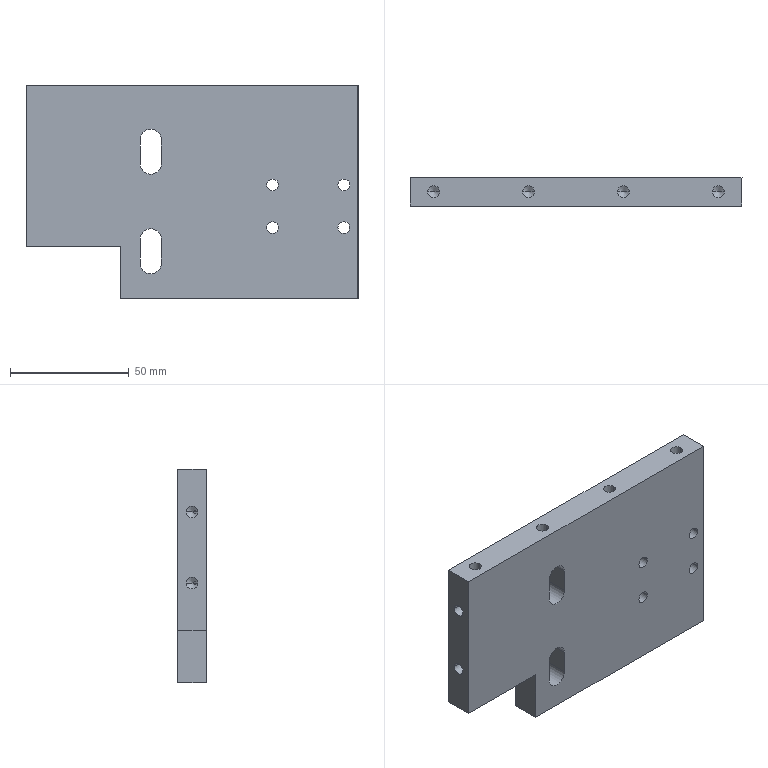Component | SolidWorks | 17081801-804-012A-1 | 1 solid | 72 faces | box 140 x 12 x 90 mm | volume 132790 mm3 | cylinder 36 | cone 24 | plane 12 | commonest cylinder face diameters 5 x32 9 x4 | material Q235
build123d program:
from build123d import *

# Parameters (mm, degrees)
SKETCH1_W                     = 12
SKETCH1_H                     = 90
BOSS_EXTRUDE1_DEPTH           = 40
SKETCH4_W                     = 12
SKETCH4_H                     = 68
BOSS_EXTRUDE2_DEPTH           = 60
M6_TAPPED_HOLE1_D             = 5
M6_TAPPED_HOLE1_DEPTH         = 13
M6_TAPPED_HOLE1_TIP           = 1.502
M6_TAPPED_HOLE2_D             = 5
M6_TAPPED_HOLE2_DEPTH         = 13
M6_TAPPED_HOLE2_TIP           = 1.502
SKETCH10_W                    = 12
SKETCH10_H                    = 22
BOSS_EXTRUDE3_DEPTH           = 20
CUT_EXTRUDE1_DEPTH            = 136.07
M6_TAPPED_HOLE3_D             = 5
M6_TAPPED_HOLE3_DEPTH         = 15
M6_TAPPED_HOLE3_TIP           = 1.502
SIZE_MM_DOWEL_PIN_HOLE1_D     = 5
SIZE_MM_DOWEL_PIN_HOLE1_DEPTH = 10
SIZE_MM_DOWEL_PIN_HOLE1_TIP   = 1.502
M6_TAPPED_HOLE4_D             = 5
M6_TAPPED_HOLE4_DEPTH         = 15
M6_TAPPED_HOLE4_TIP           = 1.502


with BuildPart() as part:
    # Sketch1 → Boss-Extrude1 (new, symmetric)
    with BuildSketch(Plane.XY):
        with Locations((0, 45)):
            Rectangle(SKETCH1_W, SKETCH1_H)
    extrude(amount=BOSS_EXTRUDE1_DEPTH, both=True)

    # Sketch4 → Boss-Extrude2 (add)
    with BuildSketch(Plane(origin=(0, 0, -40), x_dir=(-1, 0, 0), z_dir=(0, 0, -1))):
        with Locations((0, 56)):
            Rectangle(SKETCH4_W, SKETCH4_H)
    extrude(amount=BOSS_EXTRUDE2_DEPTH)

    # M6 Tapped Hole1
    with Locations(Plane(origin=(0, 90, 0), x_dir=(1, 0, 0), z_dir=(0, 1, 0))):
        with Locations((0, -30), (0, 10), (0, 50), (0, 90)):
            Hole(M6_TAPPED_HOLE1_D / 2, depth=M6_TAPPED_HOLE1_DEPTH)
            with Locations((0, 0, -(M6_TAPPED_HOLE1_DEPTH + M6_TAPPED_HOLE1_TIP / 2))):  # 118° drill point
                Cone(0, M6_TAPPED_HOLE1_D / 2, M6_TAPPED_HOLE1_TIP, mode=Mode.SUBTRACT)

    # M6 Tapped Hole2
    with Locations(Plane(origin=(0, 0, -100), x_dir=(-1, 0, 0), z_dir=(0, 0, -1))):
        with Locations((0, 42), (0, 72)):
            Hole(M6_TAPPED_HOLE2_D / 2, depth=M6_TAPPED_HOLE2_DEPTH)
            with Locations((0, 0, -(M6_TAPPED_HOLE2_DEPTH + M6_TAPPED_HOLE2_TIP / 2))):  # 118° drill point
                Cone(0, M6_TAPPED_HOLE2_D / 2, M6_TAPPED_HOLE2_TIP, mode=Mode.SUBTRACT)

    # Sketch10 → Boss-Extrude3 (add)
    with BuildSketch(Plane(origin=(0, 0, -40), x_dir=(-1, 0, 0), z_dir=(0, 0, -1))):
        with Locations((0, 11)):
            Rectangle(SKETCH10_W, SKETCH10_H)
    extrude(amount=BOSS_EXTRUDE3_DEPTH)

    # Sketch11 → Cut-Extrude1 (cut, through all)
    with BuildSketch(Plane(origin=(6, 0, 0), x_dir=(0, 0, -1), z_dir=(1, 0, 0))):
        with BuildLine():
            Line((42.9, 15), (42.9, 25))
            ThreePointArc((42.9, 25), (47.4, 29.5), (51.9, 25))
            Line((51.9, 25), (51.9, 15))
            ThreePointArc((51.9, 15), (47.4, 10.5), (42.9, 15))
        make_face()
        with BuildLine():
            Line((42.9, 57), (42.9, 67))
            ThreePointArc((42.9, 67), (47.4, 71.5), (51.9, 67))
            Line((51.9, 67), (51.9, 57))
            ThreePointArc((51.9, 57), (47.4, 52.5), (42.9, 57))
        make_face()
    extrude(amount=-CUT_EXTRUDE1_DEPTH, mode=Mode.SUBTRACT)

    # M6 Tapped Hole3
    with Locations(Plane(origin=(0, 0, 0), x_dir=(-1, 0, 0), z_dir=(0, -1, 0))):
        with Locations((0, -35), (0, -15), (0, 15), (0, 35)):
            Hole(M6_TAPPED_HOLE3_D / 2, depth=M6_TAPPED_HOLE3_DEPTH)
            with Locations((0, 0, -(M6_TAPPED_HOLE3_DEPTH + M6_TAPPED_HOLE3_TIP / 2))):  # 118° drill point
                Cone(0, M6_TAPPED_HOLE3_D / 2, M6_TAPPED_HOLE3_TIP, mode=Mode.SUBTRACT)

    # Size mm Dowel Pin Hole1
    with Locations(Plane(origin=(0, 0, 0), x_dir=(-1, 0, 0), z_dir=(0, -1, 0))):
        with Locations((0, 25), (0, -25)):
            Hole(SIZE_MM_DOWEL_PIN_HOLE1_D / 2, depth=SIZE_MM_DOWEL_PIN_HOLE1_DEPTH)
            with Locations((0, 0, -(SIZE_MM_DOWEL_PIN_HOLE1_DEPTH + SIZE_MM_DOWEL_PIN_HOLE1_TIP / 2))):  # 118° drill point
                Cone(0, SIZE_MM_DOWEL_PIN_HOLE1_D / 2, SIZE_MM_DOWEL_PIN_HOLE1_TIP, mode=Mode.SUBTRACT)

    # M6 Tapped Hole4
    with Locations(Plane.ZY.offset(6)):
        with Locations((4, 30), (34, 30), (4, 48), (34, 48)):
            Hole(M6_TAPPED_HOLE4_D / 2, depth=M6_TAPPED_HOLE4_DEPTH)
            with Locations((0, 0, -(M6_TAPPED_HOLE4_DEPTH + M6_TAPPED_HOLE4_TIP / 2))):  # 118° drill point
                Cone(0, M6_TAPPED_HOLE4_D / 2, M6_TAPPED_HOLE4_TIP, mode=Mode.SUBTRACT)


solid = part.part

# Placed as in the assembly
solid = solid.moved(Location((-14.5, 2094.4, 132), (90, 90, 0)))